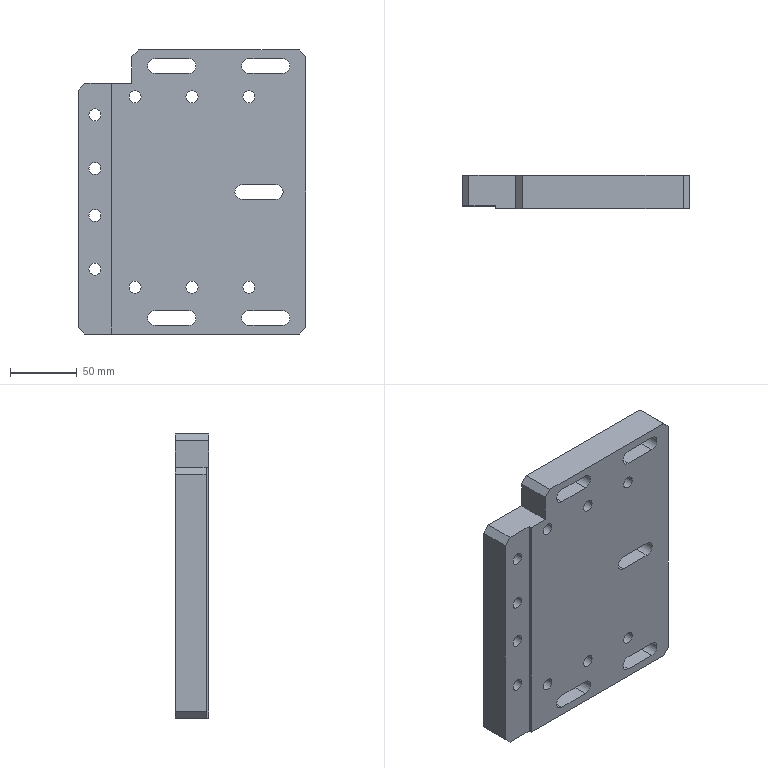Component | SolidWorks | F2-1 | 1 solid | 92 faces | box 170 x 25 x 212 mm | volume 793813 mm3 | cylinder 57 | plane 35 | commonest cylinder face diameters 15 x20 9 x20 11 x15 6.8 x2
build123d program:
from build123d import *

# Parameters (mm, degrees)
SKETCH1_W                                       = 170
SKETCH1_H                                       = 212
BOSS_EXTRUDE1_DEPTH                             = 25
SKETCH2_W                                       = 25
SKETCH2_H                                       = 2
CUT_EXTRUDE1_DEPTH                              = 536.922
SKETCH3_W                                       = 40
SKETCH3_H                                       = 25
CUT_EXTRUDE2_DEPTH                              = 513.281
CUT_EXTRUDE3_DEPTH                              = 513.281
M8_HEX_SOCKET_HEAD_CAP_SCREW_CBORE1_D           = 9
M8_HEX_SOCKET_HEAD_CAP_SCREW_CBORE1_CBORE_D     = 15
M8_HEX_SOCKET_HEAD_CAP_SCREW_CBORE1_CBORE_DEPTH = 8
M8_HEX_SOCKET_HEAD_CAP_SCREW_CBORE2_D           = 9
M8_HEX_SOCKET_HEAD_CAP_SCREW_CBORE2_CBORE_D     = 15
M8_HEX_SOCKET_HEAD_CAP_SCREW_CBORE2_CBORE_DEPTH = 8
M8_TAPPED_HOLE1_D                               = 6.8
M8_TAPPED_HOLE1_DEPTH                           = 20
M8_TAPPED_HOLE1_TIP                             = 2.043
CHAMFER1_SIZE                                   = 5


with BuildPart() as part:
    # Sketch1 → Boss-Extrude1 (new body)
    with BuildSketch(Plane.XY):
        with Locations((406.572, -36)):
            Rectangle(SKETCH1_W, SKETCH1_H)
    extrude(amount=BOSS_EXTRUDE1_DEPTH)

    # Sketch2 → Cut-Extrude1 (cut, through all)
    with BuildSketch(Plane(origin=(0, 70, 0), x_dir=(1, 0, 0), z_dir=(0, 1, 0))):
        with Locations((334.072, -1)):
            Rectangle(SKETCH2_W, SKETCH2_H)
    extrude(amount=-CUT_EXTRUDE1_DEPTH, mode=Mode.SUBTRACT)

    # Sketch3 → Cut-Extrude2 (cut, through all)
    with BuildSketch(Plane(origin=(0, 0, 0), x_dir=(-1, 0, 0), z_dir=(0, 0, -1))):
        with Locations((-341.572, -129.5)):
            Rectangle(SKETCH3_W, SKETCH3_H)
    extrude(amount=-CUT_EXTRUDE2_DEPTH, mode=Mode.SUBTRACT)

    # Sketch4 → Cut-Extrude3 (cut, through all)
    with BuildSketch(Plane(origin=(0, 0, 0), x_dir=(-1, 0, 0), z_dir=(0, 0, -1))):
        with BuildLine():
            Line((-379.072, -135.5), (-404.072, -135.5))
            ThreePointArc((-404.072, -135.5), (-409.572, -130), (-404.072, -124.5))
            Line((-404.072, -124.5), (-379.072, -124.5))
            ThreePointArc((-379.072, -124.5), (-373.572, -130), (-379.072, -135.5))
        make_face()
        with BuildLine():
            Line((-449.072, -135.5), (-474.072, -135.5))
            ThreePointArc((-474.072, -135.5), (-479.572, -130), (-474.072, -124.5))
            Line((-474.072, -124.5), (-449.072, -124.5))
            ThreePointArc((-449.072, -124.5), (-443.572, -130), (-449.072, -135.5))
        make_face()
        with BuildLine():
            Line((-444.072, -41.5), (-469.072, -41.5))
            ThreePointArc((-469.072, -41.5), (-474.572, -36), (-469.072, -30.5))
            Line((-469.072, -30.5), (-444.072, -30.5))
            ThreePointArc((-444.072, -30.5), (-438.572, -36), (-444.072, -41.5))
        make_face()
        with BuildLine():
            Line((-379.072, 63.5), (-404.072, 63.5))
            ThreePointArc((-404.072, 63.5), (-409.572, 58), (-404.072, 52.5))
            Line((-404.072, 52.5), (-379.072, 52.5))
            ThreePointArc((-379.072, 52.5), (-373.572, 58), (-379.072, 63.5))
        make_face()
        with BuildLine():
            Line((-449.072, 63.5), (-474.072, 63.5))
            ThreePointArc((-474.072, 63.5), (-479.572, 58), (-474.072, 52.5))
            Line((-474.072, 52.5), (-449.072, 52.5))
            ThreePointArc((-449.072, 52.5), (-443.572, 58), (-449.072, 63.5))
        make_face()
    extrude(amount=-CUT_EXTRUDE3_DEPTH, mode=Mode.SUBTRACT)

    # M8 Hex Socket Head Cap Screw CBORE1 (through all)
    with Locations(Plane.XY.offset(25)):
        with Locations((364.072, 35), (449.072, 35), (406.572, 35), (449.072, -107), (406.572, -107), (364.072, -107)):
            CounterBoreHole(M8_HEX_SOCKET_HEAD_CAP_SCREW_CBORE1_D / 2, M8_HEX_SOCKET_HEAD_CAP_SCREW_CBORE1_CBORE_D / 2, M8_HEX_SOCKET_HEAD_CAP_SCREW_CBORE1_CBORE_DEPTH)

    # M8 Hex Socket Head Cap Screw CBORE2 (through all)
    with Locations(Plane.XY.offset(25)):
        with Locations((334.072, -93.5), (334.072, -53.5), (334.072, 21.5), (334.072, -18.5)):
            CounterBoreHole(M8_HEX_SOCKET_HEAD_CAP_SCREW_CBORE2_D / 2, M8_HEX_SOCKET_HEAD_CAP_SCREW_CBORE2_CBORE_D / 2, M8_HEX_SOCKET_HEAD_CAP_SCREW_CBORE2_CBORE_DEPTH)

    # M8 Tapped Hole1
    with Locations(Plane(origin=(491.572, 0, 0), x_dir=(0, 0, -1), z_dir=(1, 0, 0))):
        with Locations((-12.5, -36)):
            Hole(M8_TAPPED_HOLE1_D / 2, depth=M8_TAPPED_HOLE1_DEPTH)
            with Locations((0, 0, -(M8_TAPPED_HOLE1_DEPTH + M8_TAPPED_HOLE1_TIP / 2))):  # 118° drill point
                Cone(0, M8_TAPPED_HOLE1_D / 2, M8_TAPPED_HOLE1_TIP, mode=Mode.SUBTRACT)

    # Chamfer1
    chamfer1_edges = [part.edges().sort_by_distance(p)[0] for p in [
        (321.572, -117, 13.5),
        (361.572, -142, 12.5),
        (321.572, 70, 13.5),
        (491.572, 70, 12.5),
        (491.572, -142, 12.5),
    ]]
    chamfer(chamfer1_edges, length=CHAMFER1_SIZE)


solid = part.part

# Placed as in the assembly
solid = solid.moved(Location((-225.572, 592.279, -92), (-90, 0, 0)))